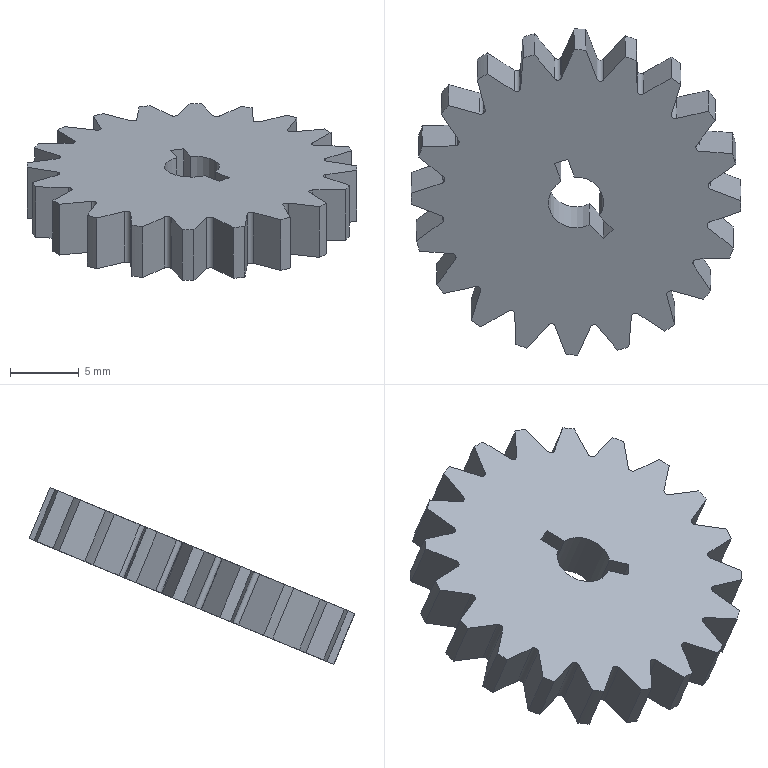Component | SolidWorks | Simple Gear-1 | 1 solid | 97 faces | box 24 x 23.71 x 12.86 mm | volume 1448 mm3 | cylinder 49 | plane 48 | commonest cylinder face diameters 0.6 x27 24 x20 4 x2
build123d program:
from build123d import *

# Parameters (mm, degrees)
BOSS_EXTRUDE1_DEPTH           = 5
SCALE1_SCALE                  = 0.4
KEYWAYRELIEF_SIMPLEGEAR_DEPTH = 10


with BuildPart() as part:
    # Sketch2 → Boss-Extrude1 (new, symmetric)
    with BuildSketch(Plane(origin=(0, 0, 0), x_dir=(1, 0, 0), z_dir=(0, 1, 0))):
        with BuildLine():
            Line((-0.6495, 24.63), (-3.623, 29.78))
            ThreePointArc((-3.623, 29.78), (-4.693, 29.631), (-5.757, 29.442))
            Line((-5.757, 29.442), (-6.993, 23.625))
            ThreePointArc((-6.993, 23.625), (-7.495, 23.068), (-8.229, 23.224))
            Line((-8.229, 23.224), (-12.649, 27.203))
            ThreePointArc((-12.649, 27.203), (-13.62, 26.73), (-14.573, 26.223))
            Line((-14.573, 26.223), (-13.952, 20.308))
            ThreePointArc((-13.952, 20.308), (-14.257, 19.623), (-15.003, 19.544))
            Line((-15.003, 19.544), (-20.436, 21.963))
            ThreePointArc((-20.436, 21.963), (-21.213, 21.213), (-21.963, 20.436))
            Line((-21.963, 20.436), (-19.544, 15.003))
            ThreePointArc((-19.544, 15.003), (-19.623, 14.257), (-20.308, 13.952))
            Line((-20.308, 13.952), (-26.223, 14.573))
            ThreePointArc((-26.223, 14.573), (-26.73, 13.62), (-27.203, 12.649))
            Line((-27.203, 12.649), (-23.224, 8.229))
            ThreePointArc((-23.224, 8.229), (-23.068, 7.495), (-23.625, 6.993))
            Line((-23.625, 6.993), (-29.442, 5.757))
            ThreePointArc((-29.442, 5.757), (-29.631, 4.693), (-29.78, 3.623))
            Line((-29.78, 3.623), (-24.63, 0.6495))
            ThreePointArc((-24.63, 0.6495), (-24.255, 0), (-24.63, -0.6495))
            Line((-24.63, -0.6495), (-29.78, -3.623))
            ThreePointArc((-29.78, -3.623), (-29.631, -4.693), (-29.442, -5.757))
            Line((-29.442, -5.757), (-23.625, -6.993))
            ThreePointArc((-23.625, -6.993), (-23.068, -7.495), (-23.224, -8.229))
            Line((-23.224, -8.229), (-27.203, -12.649))
            ThreePointArc((-27.203, -12.649), (-26.73, -13.62), (-26.223, -14.573))
            Line((-26.223, -14.573), (-20.308, -13.952))
            ThreePointArc((-20.308, -13.952), (-19.623, -14.257), (-19.544, -15.003))
            Line((-19.544, -15.003), (-21.963, -20.436))
            ThreePointArc((-21.963, -20.436), (-21.213, -21.213), (-20.436, -21.963))
            Line((-20.436, -21.963), (-15.003, -19.544))
            ThreePointArc((-15.003, -19.544), (-14.257, -19.623), (-13.952, -20.308))
            Line((-13.952, -20.308), (-14.573, -26.223))
            ThreePointArc((-14.573, -26.223), (-13.62, -26.73), (-12.649, -27.203))
            Line((-12.649, -27.203), (-8.229, -23.224))
            ThreePointArc((-8.229, -23.224), (-7.495, -23.068), (-6.993, -23.625))
            Line((-6.993, -23.625), (-5.757, -29.442))
            ThreePointArc((-5.757, -29.442), (-4.693, -29.631), (-3.623, -29.78))
            Line((-3.623, -29.78), (-0.6495, -24.63))
            ThreePointArc((-0.6495, -24.63), (0, -24.255), (0.6495, -24.63))
            Line((0.6495, -24.63), (3.623, -29.78))
            ThreePointArc((3.623, -29.78), (4.693, -29.631), (5.757, -29.442))
            Line((5.757, -29.442), (6.993, -23.625))
            ThreePointArc((6.993, -23.625), (7.495, -23.068), (8.229, -23.224))
            Line((8.229, -23.224), (12.649, -27.203))
            ThreePointArc((12.649, -27.203), (13.62, -26.73), (14.573, -26.223))
            Line((14.573, -26.223), (13.952, -20.308))
            ThreePointArc((13.952, -20.308), (14.257, -19.623), (15.003, -19.544))
            Line((15.003, -19.544), (20.436, -21.963))
            ThreePointArc((20.436, -21.963), (21.213, -21.213), (21.963, -20.436))
            Line((21.963, -20.436), (19.544, -15.003))
            ThreePointArc((19.544, -15.003), (19.623, -14.257), (20.308, -13.952))
            Line((20.308, -13.952), (26.223, -14.573))
            ThreePointArc((26.223, -14.573), (26.73, -13.62), (27.203, -12.649))
            Line((27.203, -12.649), (23.224, -8.229))
            ThreePointArc((23.224, -8.229), (23.068, -7.495), (23.625, -6.993))
            Line((23.625, -6.993), (29.442, -5.757))
            ThreePointArc((29.442, -5.757), (29.631, -4.693), (29.78, -3.623))
            Line((29.78, -3.623), (24.63, -0.6495))
            ThreePointArc((24.63, -0.6495), (24.255, 0), (24.63, 0.6495))
            Line((24.63, 0.6495), (29.78, 3.623))
            ThreePointArc((29.78, 3.623), (29.631, 4.693), (29.442, 5.757))
            Line((29.442, 5.757), (23.625, 6.993))
            ThreePointArc((23.625, 6.993), (23.068, 7.495), (23.224, 8.229))
            Line((23.224, 8.229), (27.203, 12.649))
            ThreePointArc((27.203, 12.649), (26.73, 13.62), (26.223, 14.573))
            Line((26.223, 14.573), (20.308, 13.952))
            ThreePointArc((20.308, 13.952), (19.623, 14.257), (19.544, 15.003))
            Line((19.544, 15.003), (21.963, 20.436))
            ThreePointArc((21.963, 20.436), (21.213, 21.213), (20.436, 21.963))
            Line((20.436, 21.963), (15.003, 19.544))
            ThreePointArc((15.003, 19.544), (14.257, 19.623), (13.952, 20.308))
            Line((13.952, 20.308), (14.573, 26.223))
            ThreePointArc((14.573, 26.223), (13.62, 26.73), (12.649, 27.203))
            Line((12.649, 27.203), (8.229, 23.224))
            ThreePointArc((8.229, 23.224), (7.495, 23.068), (6.993, 23.625))
            Line((6.993, 23.625), (5.757, 29.442))
            ThreePointArc((5.757, 29.442), (4.693, 29.631), (3.623, 29.78))
            Line((3.623, 29.78), (0.6495, 24.63))
            ThreePointArc((0.6495, 24.63), (0, 24.255), (-0.6495, 24.63))
        make_face()
        with BuildLine():
            Line((-1.25, 4.841), (-1.25, 8.5))
            Line((-1.25, 8.5), (1.25, 8.5))
            Line((1.25, 8.5), (1.25, 4.841))
            ThreePointArc((1.25, 4.841), (3.953, 3.062), (5, 0))
            ThreePointArc((5, 0), (-3.062, -3.953), (-1.25, 4.841))
        make_face(mode=Mode.SUBTRACT)
    extrude(amount=BOSS_EXTRUDE1_DEPTH, both=True)


with BuildPart() as part_1:
    # Scale1: scaled about (0, 0, 0)
    add(part.part.scale(SCALE1_SCALE))

    # Sketch3 → KeywayRelief_SimpleGear (cut, symmetric)
    with BuildSketch(Plane(origin=(0, 0, 0), x_dir=(1, 0, 0), z_dir=(0, 1, 0))):
        Polygon((0.7169, -0.3258), (1.909, -2.859), (0.9859, -3.294), (-0.2061, -0.76), align=None)
    extrude(amount=KEYWAYRELIEF_SIMPLEGEAR_DEPTH, both=True, mode=Mode.SUBTRACT)


solid = part_1.part

# Placed as in the assembly
solid = solid.moved(Location((320.621, -1.715, 67.15), (-67.552, -43.62, 0)))